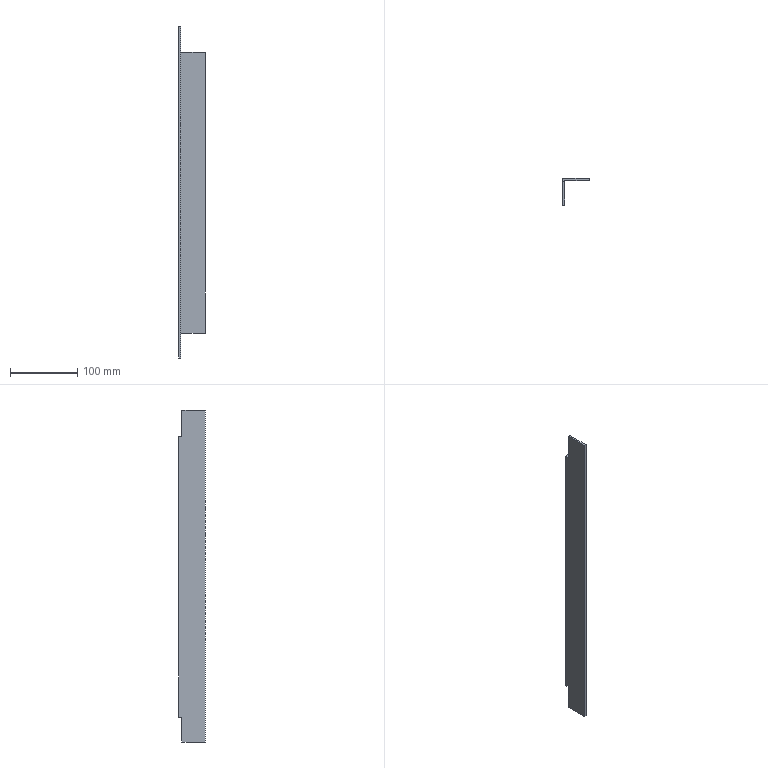Component | SolidWorks | LX-TSJ-14-1 | 1 solid | 12 faces | box 40 x 40 x 494 mm | volume 104538 mm3 | plane 12
STEP:
#1=COLOUR_RGB('',0.7922,0.8196,0.9333);
#2=FILL_AREA_STYLE_COLOUR('',#1);
#3=FILL_AREA_STYLE('',(#2));
#4=SURFACE_STYLE_FILL_AREA(#3);
#5=SURFACE_SIDE_STYLE('',(#4));
#6=SURFACE_STYLE_USAGE(.BOTH.,#5);
#7=PRESENTATION_STYLE_ASSIGNMENT((#6));
#8=CARTESIAN_POINT('',(-3.988,-23.756,-24.579));
#9=VERTEX_POINT('',#8);
#10=CARTESIAN_POINT('',(-3.988,-23.756,-26.035));
#11=VERTEX_POINT('',#10);
#12=CARTESIAN_POINT('',(-3.988,-23.756,-26.035));
#13=DIRECTION('',(-0.,0.,-1.));
#14=VECTOR('',#13,39.37);
#15=LINE('',#12,#14);
#16=EDGE_CURVE('',#9,#11,#15,.T.);
#17=ORIENTED_EDGE('',*,*,#16,.F.);
#18=CARTESIAN_POINT('',(-3.988,-23.678,-24.579));
#19=VERTEX_POINT('',#18);
#20=CARTESIAN_POINT('',(-3.988,-25.134,-24.579));
#21=DIRECTION('',(0.,-1.,-0.));
#22=VECTOR('',#21,39.37);
#23=LINE('',#20,#22);
#24=EDGE_CURVE('',#19,#9,#23,.T.);
#25=ORIENTED_EDGE('',*,*,#24,.F.);
#26=CARTESIAN_POINT('',(-3.988,-23.678,-8.122));
#27=VERTEX_POINT('',#26);
#28=CARTESIAN_POINT('',(-3.988,-23.678,-6.587));
#29=DIRECTION('',(0.,0.,1.));
#30=VECTOR('',#29,39.37);
#31=LINE('',#28,#30);
#32=EDGE_CURVE('',#19,#27,#31,.T.);
#33=ORIENTED_EDGE('',*,*,#32,.T.);
#34=CARTESIAN_POINT('',(-3.988,-23.756,-8.122));
#35=VERTEX_POINT('',#34);
#36=CARTESIAN_POINT('',(-3.988,-23.756,-8.122));
#37=DIRECTION('',(0.,-1.,-0.));
#38=VECTOR('',#37,39.37);
#39=LINE('',#36,#38);
#40=EDGE_CURVE('',#27,#35,#39,.T.);
#41=ORIENTED_EDGE('',*,*,#40,.T.);
#42=CARTESIAN_POINT('',(-3.988,-23.756,-6.587));
#43=VERTEX_POINT('',#42);
#44=CARTESIAN_POINT('',(-3.988,-23.756,-26.035));
#45=DIRECTION('',(0.,0.,1.));
#46=VECTOR('',#45,39.37);
#47=LINE('',#44,#46);
#48=EDGE_CURVE('',#35,#43,#47,.T.);
#49=ORIENTED_EDGE('',*,*,#48,.T.);
#50=CARTESIAN_POINT('',(-3.988,-25.134,-6.587));
#51=VERTEX_POINT('',#50);
#52=CARTESIAN_POINT('',(-3.988,-25.134,-6.587));
#53=DIRECTION('',(-0.,1.,0.));
#54=VECTOR('',#53,39.37);
#55=LINE('',#52,#54);
#56=EDGE_CURVE('',#51,#43,#55,.T.);
#57=ORIENTED_EDGE('',*,*,#56,.F.);
#58=CARTESIAN_POINT('',(-3.988,-25.134,-26.035));
#59=VERTEX_POINT('',#58);
#60=CARTESIAN_POINT('',(-3.988,-25.134,-6.587));
#61=DIRECTION('',(-0.,0.,-1.));
#62=VECTOR('',#61,39.37);
#63=LINE('',#60,#62);
#64=EDGE_CURVE('',#51,#59,#63,.T.);
#65=ORIENTED_EDGE('',*,*,#64,.T.);
#66=CARTESIAN_POINT('',(-3.988,-25.134,-26.035));
#67=DIRECTION('',(-0.,1.,0.));
#68=VECTOR('',#67,39.37);
#69=LINE('',#66,#68);
#70=EDGE_CURVE('',#59,#11,#69,.T.);
#71=ORIENTED_EDGE('',*,*,#70,.T.);
#72=EDGE_LOOP('',(#17,#25,#33,#41,#49,#57,#65,#71));
#73=FACE_OUTER_BOUND('',#72,.T.);
#74=CARTESIAN_POINT('',(-3.988,-25.134,-6.587));
#75=DIRECTION('',(-1.,-0.,0.));
#76=DIRECTION('',(0.,0.,1.));
#77=AXIS2_PLACEMENT_3D('',#74,#75,#76);
#78=PLANE('',#77);
#79=ADVANCED_FACE('',(#73),#78,.F.);
#80=CARTESIAN_POINT('',(-2.531,-23.678,-24.579));
#81=VERTEX_POINT('',#80);
#82=CARTESIAN_POINT('',(-3.988,-23.678,-24.579));
#83=DIRECTION('',(-1.,-0.,0.));
#84=VECTOR('',#83,39.37);
#85=LINE('',#82,#84);
#86=EDGE_CURVE('',#81,#19,#85,.T.);
#87=ORIENTED_EDGE('',*,*,#86,.F.);
#88=CARTESIAN_POINT('',(-2.531,-23.678,-8.122));
#89=VERTEX_POINT('',#88);
#90=CARTESIAN_POINT('',(-2.531,-23.678,-6.587));
#91=DIRECTION('',(0.,0.,1.));
#92=VECTOR('',#91,39.37);
#93=LINE('',#90,#92);
#94=EDGE_CURVE('',#81,#89,#93,.T.);
#95=ORIENTED_EDGE('',*,*,#94,.T.);
#96=CARTESIAN_POINT('',(-2.531,-23.678,-8.122));
#97=DIRECTION('',(-1.,-0.,0.));
#98=VECTOR('',#97,39.37);
#99=LINE('',#96,#98);
#100=EDGE_CURVE('',#89,#27,#99,.T.);
#101=ORIENTED_EDGE('',*,*,#100,.T.);
#102=ORIENTED_EDGE('',*,*,#32,.F.);
#103=EDGE_LOOP('',(#87,#95,#101,#102));
#104=FACE_OUTER_BOUND('',#103,.T.);
#105=CARTESIAN_POINT('',(-3.988,-23.678,-6.587));
#106=DIRECTION('',(-0.,1.,0.));
#107=DIRECTION('',(-0.,0.,-1.));
#108=AXIS2_PLACEMENT_3D('',#105,#106,#107);
#109=PLANE('',#108);
#110=ADVANCED_FACE('',(#104),#109,.F.);
#111=CARTESIAN_POINT('',(-2.531,-23.56,-24.579));
#112=VERTEX_POINT('',#111);
#113=CARTESIAN_POINT('',(-2.531,-23.678,-24.579));
#114=DIRECTION('',(0.,-1.,-0.));
#115=VECTOR('',#114,39.37);
#116=LINE('',#113,#115);
#117=EDGE_CURVE('',#112,#81,#116,.T.);
#118=ORIENTED_EDGE('',*,*,#117,.F.);
#119=CARTESIAN_POINT('',(-2.531,-23.56,-8.122));
#120=VERTEX_POINT('',#119);
#121=CARTESIAN_POINT('',(-2.531,-23.56,-6.587));
#122=DIRECTION('',(0.,0.,1.));
#123=VECTOR('',#122,39.37);
#124=LINE('',#121,#123);
#125=EDGE_CURVE('',#112,#120,#124,.T.);
#126=ORIENTED_EDGE('',*,*,#125,.T.);
#127=CARTESIAN_POINT('',(-2.531,-23.756,-8.122));
#128=DIRECTION('',(0.,-1.,-0.));
#129=VECTOR('',#128,39.37);
#130=LINE('',#127,#129);
#131=EDGE_CURVE('',#120,#89,#130,.T.);
#132=ORIENTED_EDGE('',*,*,#131,.T.);
#133=ORIENTED_EDGE('',*,*,#94,.F.);
#134=EDGE_LOOP('',(#118,#126,#132,#133));
#135=FACE_OUTER_BOUND('',#134,.T.);
#136=CARTESIAN_POINT('',(-2.531,-23.678,-6.587));
#137=DIRECTION('',(-1.,-0.,0.));
#138=DIRECTION('',(0.,0.,1.));
#139=AXIS2_PLACEMENT_3D('',#136,#137,#138);
#140=PLANE('',#139);
#141=ADVANCED_FACE('',(#135),#140,.F.);
#142=CARTESIAN_POINT('',(-4.106,-23.56,-24.579));
#143=VERTEX_POINT('',#142);
#144=CARTESIAN_POINT('',(-4.106,-23.56,-24.579));
#145=DIRECTION('',(1.,0.,-0.));
#146=VECTOR('',#145,39.37);
#147=LINE('',#144,#146);
#148=EDGE_CURVE('',#143,#112,#147,.T.);
#149=ORIENTED_EDGE('',*,*,#148,.F.);
#150=CARTESIAN_POINT('',(-4.106,-23.56,-8.122));
#151=VERTEX_POINT('',#150);
#152=CARTESIAN_POINT('',(-4.106,-23.56,-6.587));
#153=DIRECTION('',(0.,0.,1.));
#154=VECTOR('',#153,39.37);
#155=LINE('',#152,#154);
#156=EDGE_CURVE('',#143,#151,#155,.T.);
#157=ORIENTED_EDGE('',*,*,#156,.T.);
#158=CARTESIAN_POINT('',(-4.106,-23.56,-8.122));
#159=DIRECTION('',(-1.,-0.,0.));
#160=VECTOR('',#159,39.37);
#161=LINE('',#158,#160);
#162=EDGE_CURVE('',#120,#151,#161,.T.);
#163=ORIENTED_EDGE('',*,*,#162,.F.);
#164=ORIENTED_EDGE('',*,*,#125,.F.);
#165=EDGE_LOOP('',(#149,#157,#163,#164));
#166=FACE_OUTER_BOUND('',#165,.T.);
#167=CARTESIAN_POINT('',(-4.106,-23.56,-6.587));
#168=DIRECTION('',(0.,-1.,-0.));
#169=DIRECTION('',(0.,0.,1.));
#170=AXIS2_PLACEMENT_3D('',#167,#168,#169);
#171=PLANE('',#170);
#172=ADVANCED_FACE('',(#166),#171,.F.);
#173=CARTESIAN_POINT('',(-4.106,-23.756,-24.579));
#174=VERTEX_POINT('',#173);
#175=CARTESIAN_POINT('',(-4.106,-25.134,-24.579));
#176=DIRECTION('',(-0.,1.,0.));
#177=VECTOR('',#176,39.37);
#178=LINE('',#175,#177);
#179=EDGE_CURVE('',#174,#143,#178,.T.);
#180=ORIENTED_EDGE('',*,*,#179,.F.);
#181=CARTESIAN_POINT('',(-4.106,-23.756,-26.035));
#182=VERTEX_POINT('',#181);
#183=CARTESIAN_POINT('',(-4.106,-23.756,-6.587));
#184=DIRECTION('',(0.,0.,1.));
#185=VECTOR('',#184,39.37);
#186=LINE('',#183,#185);
#187=EDGE_CURVE('',#182,#174,#186,.T.);
#188=ORIENTED_EDGE('',*,*,#187,.F.);
#189=CARTESIAN_POINT('',(-4.106,-25.134,-26.035));
#190=VERTEX_POINT('',#189);
#191=CARTESIAN_POINT('',(-4.106,-25.134,-26.035));
#192=DIRECTION('',(-0.,1.,0.));
#193=VECTOR('',#192,39.37);
#194=LINE('',#191,#193);
#195=EDGE_CURVE('',#190,#182,#194,.T.);
#196=ORIENTED_EDGE('',*,*,#195,.F.);
#197=CARTESIAN_POINT('',(-4.106,-25.134,-6.587));
#198=VERTEX_POINT('',#197);
#199=CARTESIAN_POINT('',(-4.106,-25.134,-6.587));
#200=DIRECTION('',(-0.,0.,-1.));
#201=VECTOR('',#200,39.37);
#202=LINE('',#199,#201);
#203=EDGE_CURVE('',#198,#190,#202,.T.);
#204=ORIENTED_EDGE('',*,*,#203,.F.);
#205=CARTESIAN_POINT('',(-4.106,-23.756,-6.587));
#206=VERTEX_POINT('',#205);
#207=CARTESIAN_POINT('',(-4.106,-25.134,-6.587));
#208=DIRECTION('',(0.,-1.,-0.));
#209=VECTOR('',#208,39.37);
#210=LINE('',#207,#209);
#211=EDGE_CURVE('',#206,#198,#210,.T.);
#212=ORIENTED_EDGE('',*,*,#211,.F.);
#213=CARTESIAN_POINT('',(-4.106,-23.756,-8.122));
#214=VERTEX_POINT('',#213);
#215=CARTESIAN_POINT('',(-4.106,-23.756,-6.587));
#216=DIRECTION('',(0.,0.,1.));
#217=VECTOR('',#216,39.37);
#218=LINE('',#215,#217);
#219=EDGE_CURVE('',#214,#206,#218,.T.);
#220=ORIENTED_EDGE('',*,*,#219,.F.);
#221=CARTESIAN_POINT('',(-4.106,-25.134,-8.122));
#222=DIRECTION('',(0.,-1.,-0.));
#223=VECTOR('',#222,39.37);
#224=LINE('',#221,#223);
#225=EDGE_CURVE('',#151,#214,#224,.T.);
#226=ORIENTED_EDGE('',*,*,#225,.F.);
#227=ORIENTED_EDGE('',*,*,#156,.F.);
#228=EDGE_LOOP('',(#180,#188,#196,#204,#212,#220,#226,#227));
#229=FACE_OUTER_BOUND('',#228,.T.);
#230=CARTESIAN_POINT('',(-4.106,-25.134,-6.587));
#231=DIRECTION('',(1.,0.,-0.));
#232=DIRECTION('',(-0.,0.,-1.));
#233=AXIS2_PLACEMENT_3D('',#230,#231,#232);
#234=PLANE('',#233);
#235=ADVANCED_FACE('',(#229),#234,.F.);
#236=ORIENTED_EDGE('',*,*,#187,.T.);
#237=CARTESIAN_POINT('',(-2.492,-23.756,-24.579));
#238=DIRECTION('',(1.,0.,-0.));
#239=VECTOR('',#238,39.37);
#240=LINE('',#237,#239);
#241=EDGE_CURVE('',#174,#9,#240,.T.);
#242=ORIENTED_EDGE('',*,*,#241,.T.);
#243=ORIENTED_EDGE('',*,*,#16,.T.);
#244=CARTESIAN_POINT('',(-4.106,-23.756,-26.035));
#245=DIRECTION('',(-1.,-0.,0.));
#246=VECTOR('',#245,39.37);
#247=LINE('',#244,#246);
#248=EDGE_CURVE('',#11,#182,#247,.T.);
#249=ORIENTED_EDGE('',*,*,#248,.T.);
#250=EDGE_LOOP('',(#236,#242,#243,#249));
#251=FACE_OUTER_BOUND('',#250,.T.);
#252=CARTESIAN_POINT('',(-4.106,-23.756,-26.035));
#253=DIRECTION('',(-0.,1.,0.));
#254=DIRECTION('',(-0.,0.,-1.));
#255=AXIS2_PLACEMENT_3D('',#252,#253,#254);
#256=PLANE('',#255);
#257=ADVANCED_FACE('',(#251),#256,.T.);
#258=ORIENTED_EDGE('',*,*,#70,.F.);
#259=CARTESIAN_POINT('',(-4.106,-25.134,-26.035));
#260=DIRECTION('',(1.,0.,-0.));
#261=VECTOR('',#260,39.37);
#262=LINE('',#259,#261);
#263=EDGE_CURVE('',#190,#59,#262,.T.);
#264=ORIENTED_EDGE('',*,*,#263,.F.);
#265=ORIENTED_EDGE('',*,*,#195,.T.);
#266=ORIENTED_EDGE('',*,*,#248,.F.);
#267=EDGE_LOOP('',(#258,#264,#265,#266));
#268=FACE_OUTER_BOUND('',#267,.T.);
#269=CARTESIAN_POINT('',(-4.106,-25.134,-26.035));
#270=DIRECTION('',(0.,-0.,1.));
#271=DIRECTION('',(-0.,1.,0.));
#272=AXIS2_PLACEMENT_3D('',#269,#270,#271);
#273=PLANE('',#272);
#274=ADVANCED_FACE('',(#268),#273,.F.);
#275=ORIENTED_EDGE('',*,*,#64,.F.);
#276=CARTESIAN_POINT('',(-4.106,-25.134,-6.587));
#277=DIRECTION('',(1.,0.,-0.));
#278=VECTOR('',#277,39.37);
#279=LINE('',#276,#278);
#280=EDGE_CURVE('',#198,#51,#279,.T.);
#281=ORIENTED_EDGE('',*,*,#280,.F.);
#282=ORIENTED_EDGE('',*,*,#203,.T.);
#283=ORIENTED_EDGE('',*,*,#263,.T.);
#284=EDGE_LOOP('',(#275,#281,#282,#283));
#285=FACE_OUTER_BOUND('',#284,.T.);
#286=CARTESIAN_POINT('',(-4.106,-25.134,-6.587));
#287=DIRECTION('',(-0.,1.,0.));
#288=DIRECTION('',(-0.,0.,-1.));
#289=AXIS2_PLACEMENT_3D('',#286,#287,#288);
#290=PLANE('',#289);
#291=ADVANCED_FACE('',(#285),#290,.F.);
#292=ORIENTED_EDGE('',*,*,#280,.T.);
#293=ORIENTED_EDGE('',*,*,#56,.T.);
#294=CARTESIAN_POINT('',(-4.106,-23.756,-6.587));
#295=DIRECTION('',(-1.,-0.,0.));
#296=VECTOR('',#295,39.37);
#297=LINE('',#294,#296);
#298=EDGE_CURVE('',#43,#206,#297,.T.);
#299=ORIENTED_EDGE('',*,*,#298,.T.);
#300=ORIENTED_EDGE('',*,*,#211,.T.);
#301=EDGE_LOOP('',(#292,#293,#299,#300));
#302=FACE_OUTER_BOUND('',#301,.T.);
#303=CARTESIAN_POINT('',(-4.106,-25.134,-6.587));
#304=DIRECTION('',(0.,-0.,1.));
#305=DIRECTION('',(-0.,1.,0.));
#306=AXIS2_PLACEMENT_3D('',#303,#304,#305);
#307=PLANE('',#306);
#308=ADVANCED_FACE('',(#302),#307,.T.);
#309=ORIENTED_EDGE('',*,*,#219,.T.);
#310=ORIENTED_EDGE('',*,*,#298,.F.);
#311=ORIENTED_EDGE('',*,*,#48,.F.);
#312=CARTESIAN_POINT('',(-4.106,-23.756,-8.122));
#313=DIRECTION('',(1.,0.,-0.));
#314=VECTOR('',#313,39.37);
#315=LINE('',#312,#314);
#316=EDGE_CURVE('',#214,#35,#315,.T.);
#317=ORIENTED_EDGE('',*,*,#316,.F.);
#318=EDGE_LOOP('',(#309,#310,#311,#317));
#319=FACE_OUTER_BOUND('',#318,.T.);
#320=CARTESIAN_POINT('',(-4.106,-23.756,-26.035));
#321=DIRECTION('',(0.,-1.,-0.));
#322=DIRECTION('',(0.,0.,1.));
#323=AXIS2_PLACEMENT_3D('',#320,#321,#322);
#324=PLANE('',#323);
#325=ADVANCED_FACE('',(#319),#324,.F.);
#326=ORIENTED_EDGE('',*,*,#225,.T.);
#327=ORIENTED_EDGE('',*,*,#316,.T.);
#328=ORIENTED_EDGE('',*,*,#40,.F.);
#329=ORIENTED_EDGE('',*,*,#100,.F.);
#330=ORIENTED_EDGE('',*,*,#131,.F.);
#331=ORIENTED_EDGE('',*,*,#162,.T.);
#332=EDGE_LOOP('',(#326,#327,#328,#329,#330,#331));
#333=FACE_OUTER_BOUND('',#332,.T.);
#334=CARTESIAN_POINT('',(-2.531,-23.756,-8.122));
#335=DIRECTION('',(-0.,0.,-1.));
#336=DIRECTION('',(0.,-1.,-0.));
#337=AXIS2_PLACEMENT_3D('',#334,#335,#336);
#338=PLANE('',#337);
#339=ADVANCED_FACE('',(#333),#338,.F.);
#340=ORIENTED_EDGE('',*,*,#24,.T.);
#341=ORIENTED_EDGE('',*,*,#241,.F.);
#342=ORIENTED_EDGE('',*,*,#179,.T.);
#343=ORIENTED_EDGE('',*,*,#148,.T.);
#344=ORIENTED_EDGE('',*,*,#117,.T.);
#345=ORIENTED_EDGE('',*,*,#86,.T.);
#346=EDGE_LOOP('',(#340,#341,#342,#343,#344,#345));
#347=FACE_OUTER_BOUND('',#346,.T.);
#348=CARTESIAN_POINT('',(-4.106,-25.134,-24.579));
#349=DIRECTION('',(-0.,0.,-1.));
#350=DIRECTION('',(0.,-1.,-0.));
#351=AXIS2_PLACEMENT_3D('',#348,#349,#350);
#352=PLANE('',#351);
#353=ADVANCED_FACE('',(#347),#352,.T.);
#354=CLOSED_SHELL('',(#79,#110,#141,#172,#235,#257,#274,#291,#308,#325,#339,#353));
#355=MANIFOLD_SOLID_BREP('',#354);
#356=STYLED_ITEM('',(#7),#355);
#357=(LENGTH_UNIT()NAMED_UNIT(*)SI_UNIT($,.METRE.));
#358=LENGTH_MEASURE_WITH_UNIT(LENGTH_MEASURE(0.0254),#357);
#359=DIMENSIONAL_EXPONENTS(1.,0.,0.,0.,0.,0.,0.);
#360=(CONVERSION_BASED_UNIT('',#358)LENGTH_UNIT()NAMED_UNIT(#359));
#361=UNCERTAINTY_MEASURE_WITH_UNIT(LENGTH_MEASURE(0.00001),#360,'','');
#362=(NAMED_UNIT(*)PLANE_ANGLE_UNIT()SI_UNIT($,.RADIAN.));
#363=(NAMED_UNIT(*)SI_UNIT($,.STERADIAN.)SOLID_ANGLE_UNIT());
#364=(GEOMETRIC_REPRESENTATION_CONTEXT(3)GLOBAL_UNCERTAINTY_ASSIGNED_CONTEXT((#361))GLOBAL_UNIT_ASSIGNED_CONTEXT((#360,#362,#363))REPRESENTATION_CONTEXT('',''));
#365=MECHANICAL_DESIGN_GEOMETRIC_PRESENTATION_REPRESENTATION('',(#356),#364);
#366=CARTESIAN_POINT('',(0.,0.,0.));
#367=DIRECTION('',(0.,0.,1.));
#368=DIRECTION('',(1.,0.,0.));
#369=AXIS2_PLACEMENT_3D('',#366,#367,#368);
#370=(LENGTH_UNIT()NAMED_UNIT(*)SI_UNIT($,.METRE.));
#371=LENGTH_MEASURE_WITH_UNIT(LENGTH_MEASURE(0.0254),#370);
#372=DIMENSIONAL_EXPONENTS(1.,0.,0.,0.,0.,0.,0.);
#373=(CONVERSION_BASED_UNIT('',#371)LENGTH_UNIT()NAMED_UNIT(#372));
#374=UNCERTAINTY_MEASURE_WITH_UNIT(LENGTH_MEASURE(0.00001),#373,'','');
#375=(NAMED_UNIT(*)PLANE_ANGLE_UNIT()SI_UNIT($,.RADIAN.));
#376=(NAMED_UNIT(*)SI_UNIT($,.STERADIAN.)SOLID_ANGLE_UNIT());
#377=(GEOMETRIC_REPRESENTATION_CONTEXT(3)GLOBAL_UNCERTAINTY_ASSIGNED_CONTEXT((#374))GLOBAL_UNIT_ASSIGNED_CONTEXT((#373,#375,#376))REPRESENTATION_CONTEXT('',''));
#378=ADVANCED_BREP_SHAPE_REPRESENTATION('',(#355,#369),#377);
#379=PRESENTATION_LAYER_ASSIGNMENT('','',(#356));